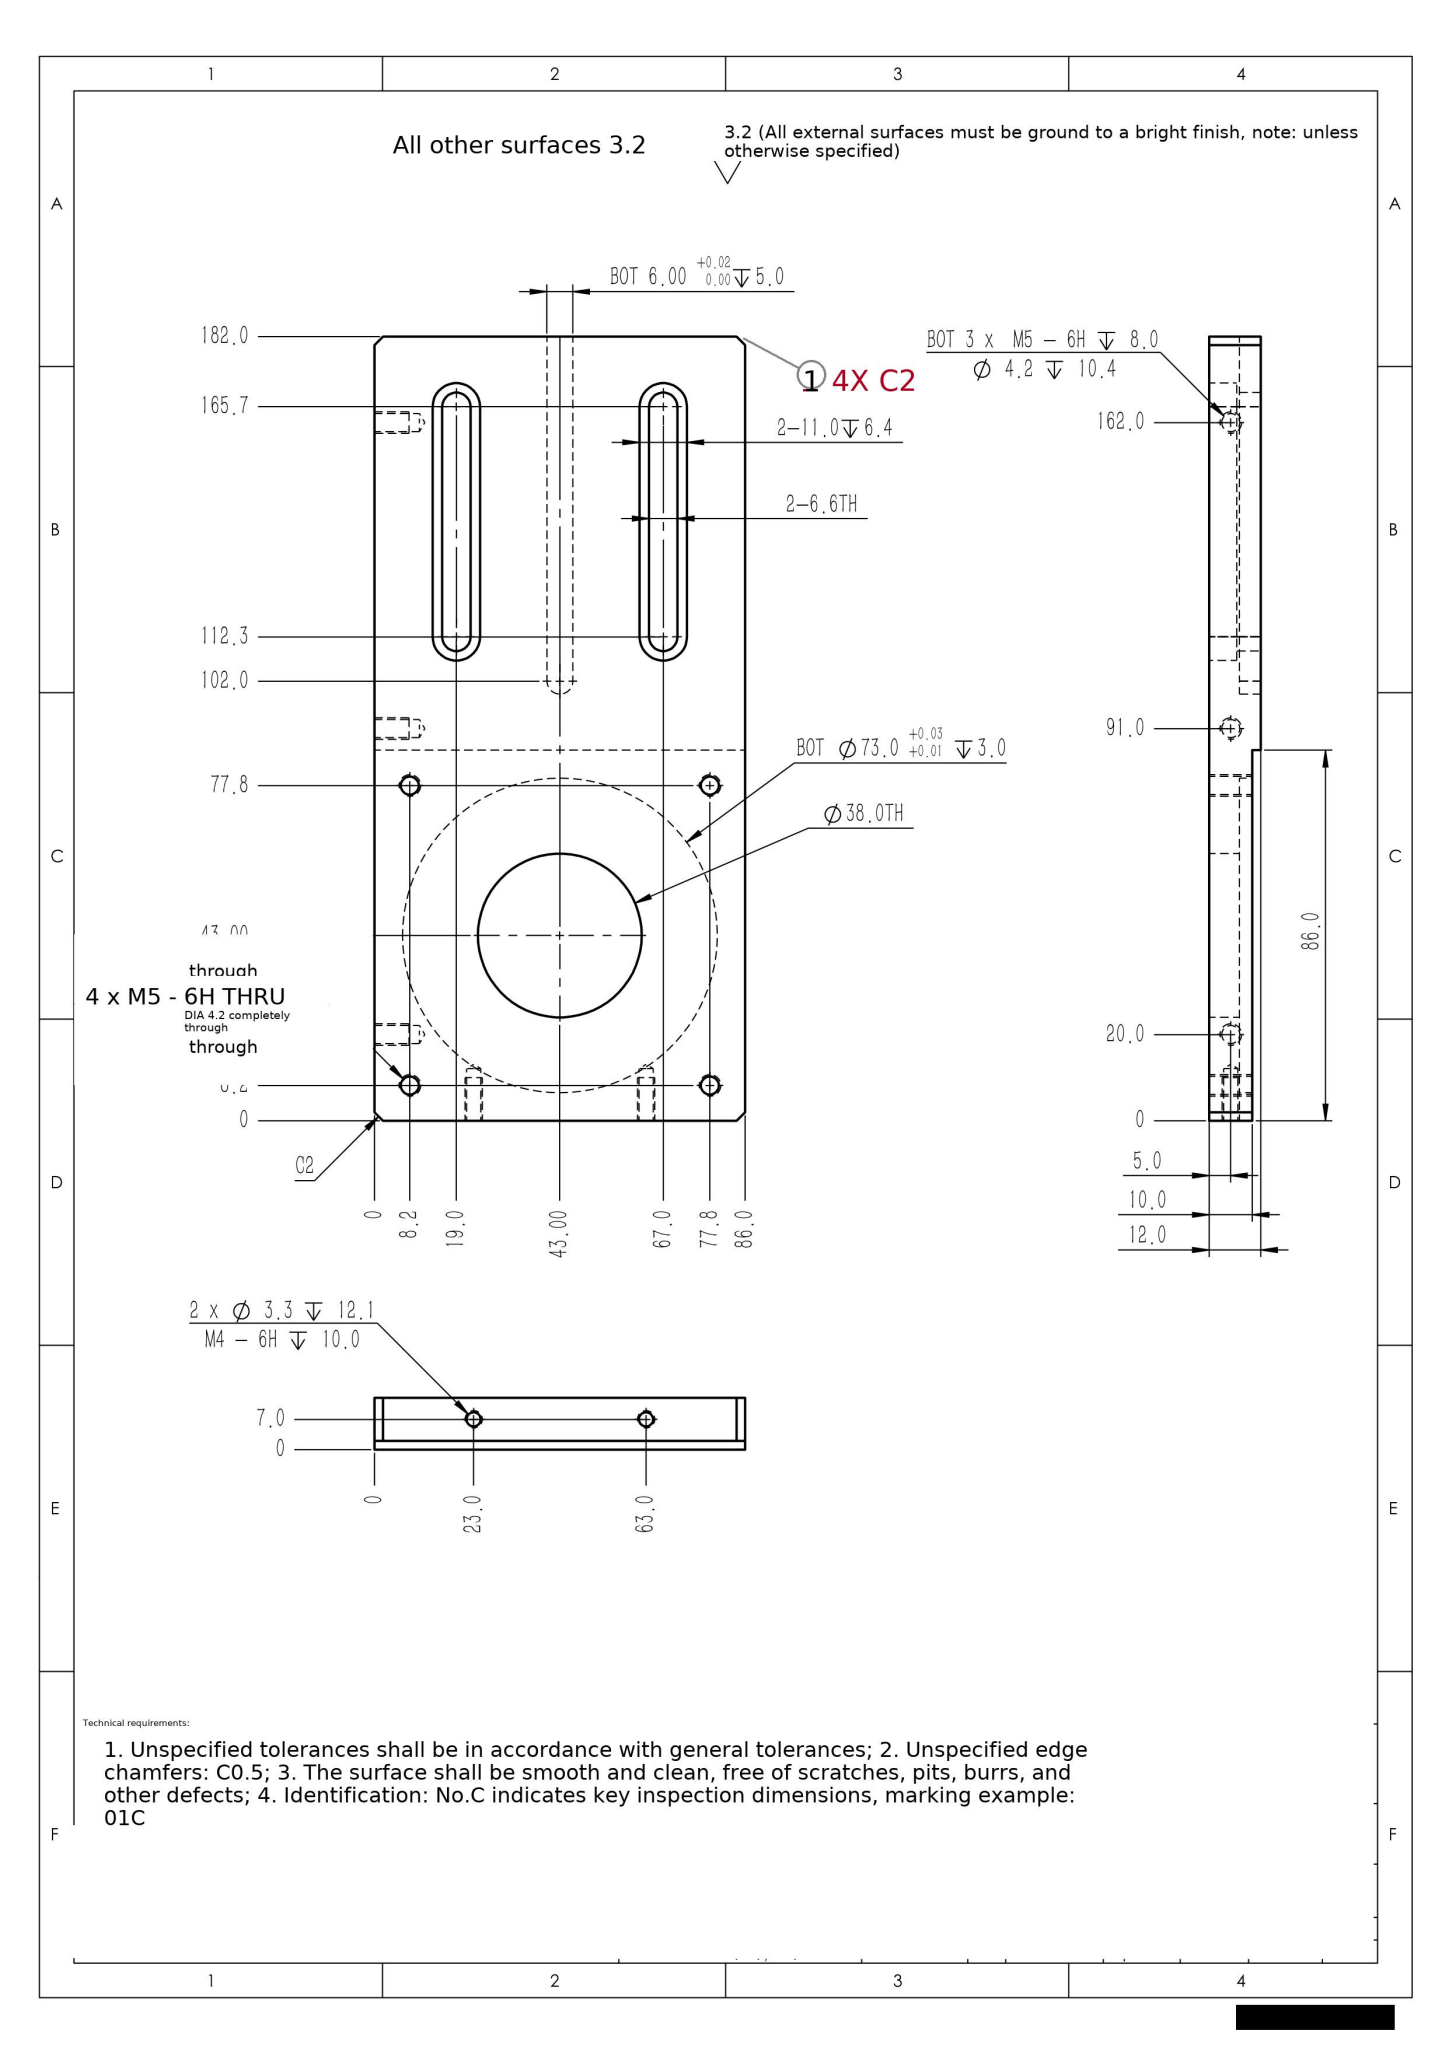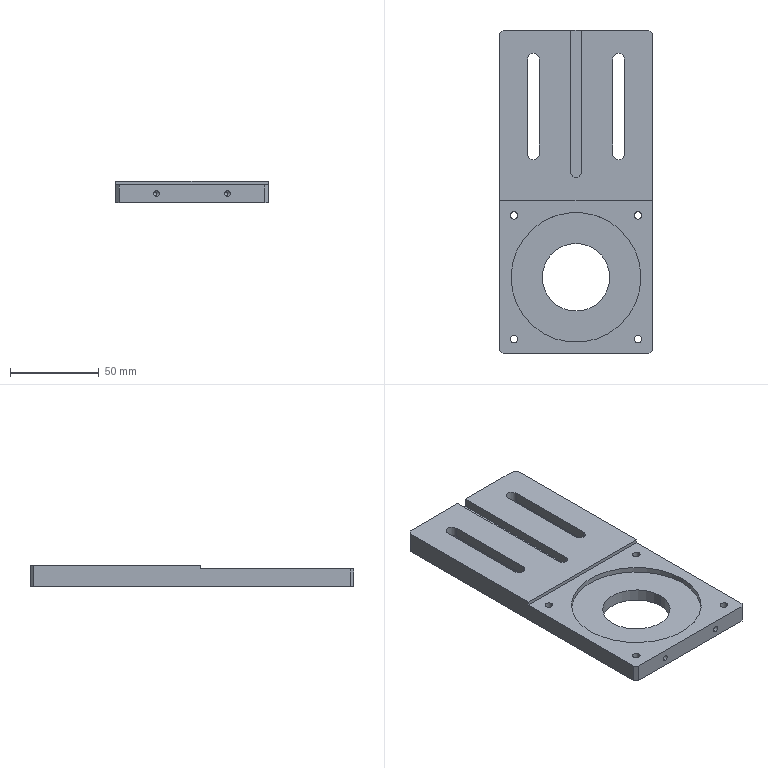Part | SolidWorks | mm | 1 solid | 67 faces | box 86 x 182 x 12 mm | volume 135696 mm3 | cylinder 31 | plane 26 | cone 10 | commonest cylinder face diameters 4.2 x14 3.3 x4 6.6 x4 11 x4 38 x2 73 x2 6 x1